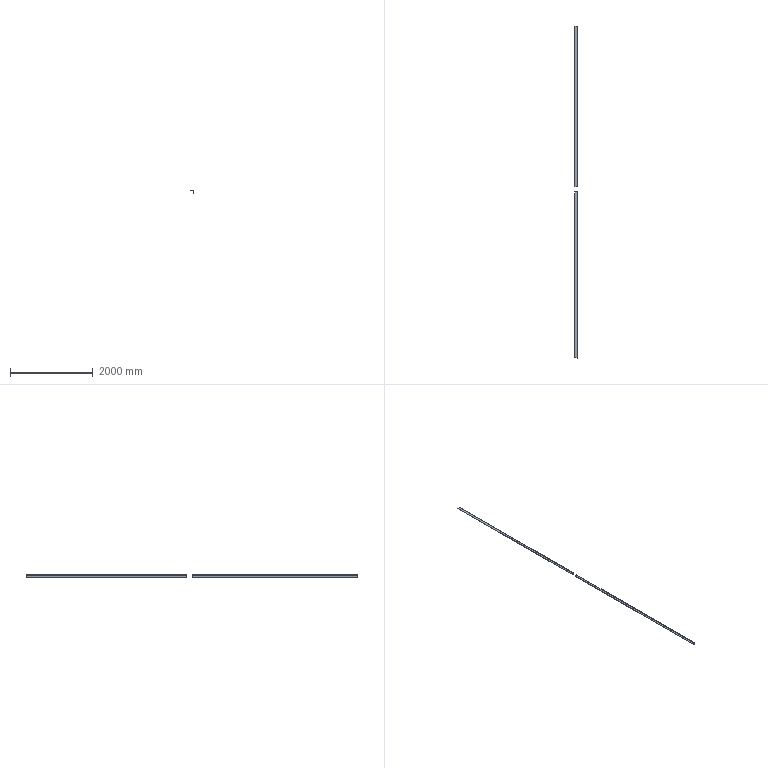Component | SolidWorks | 63#AngleIron-47 | 2 solids | 22 faces | box 63 x 8000 x 63 mm | volume 3919801 mm3 | plane 16 | cylinder 6 | commonest cylinder face diameters 2.667 x4 14 x2
STEP:
#1=CARTESIAN_POINT('',(81.493,-440.742,145.512));
#2=VERTEX_POINT('',#1);
#3=CARTESIAN_POINT('',(81.493,-598.222,145.512));
#4=VERTEX_POINT('',#3);
#5=CARTESIAN_POINT('',(81.493,-283.262,145.512));
#6=DIRECTION('',(-0.,-1.,0.));
#7=VECTOR('',#6,39.37);
#8=LINE('',#5,#7);
#9=EDGE_CURVE('',#2,#4,#8,.T.);
#10=ORIENTED_EDGE('',*,*,#9,.F.);
#11=CARTESIAN_POINT('',(81.493,-440.742,147.992));
#12=VERTEX_POINT('',#11);
#13=CARTESIAN_POINT('',(81.493,-440.742,145.512));
#14=DIRECTION('',(0.,-0.,1.));
#15=VECTOR('',#14,39.37);
#16=LINE('',#13,#15);
#17=EDGE_CURVE('',#2,#12,#16,.T.);
#18=ORIENTED_EDGE('',*,*,#17,.T.);
#19=CARTESIAN_POINT('',(81.493,-598.222,147.992));
#20=VERTEX_POINT('',#19);
#21=CARTESIAN_POINT('',(81.493,-283.262,147.992));
#22=DIRECTION('',(-0.,-1.,0.));
#23=VECTOR('',#22,39.37);
#24=LINE('',#21,#23);
#25=EDGE_CURVE('',#12,#20,#24,.T.);
#26=ORIENTED_EDGE('',*,*,#25,.T.);
#27=CARTESIAN_POINT('',(81.493,-598.222,145.512));
#28=DIRECTION('',(-0.,-0.,-1.));
#29=VECTOR('',#28,39.37);
#30=LINE('',#27,#29);
#31=EDGE_CURVE('',#20,#4,#30,.T.);
#32=ORIENTED_EDGE('',*,*,#31,.T.);
#33=EDGE_LOOP('',(#10,#18,#26,#32));
#34=FACE_OUTER_BOUND('',#33,.T.);
#35=CARTESIAN_POINT('',(81.493,-283.262,145.512));
#36=DIRECTION('',(-1.,0.,0.));
#37=DIRECTION('',(0.,1.,-0.));
#38=AXIS2_PLACEMENT_3D('',#35,#36,#37);
#39=PLANE('',#38);
#40=ADVANCED_FACE('',(#34),#39,.F.);
#41=CARTESIAN_POINT('',(81.388,-440.742,145.512));
#42=VERTEX_POINT('',#41);
#43=CARTESIAN_POINT('',(81.388,-598.222,145.512));
#44=VERTEX_POINT('',#43);
#45=CARTESIAN_POINT('',(81.388,-283.262,145.512));
#46=DIRECTION('',(-0.,-1.,0.));
#47=VECTOR('',#46,39.37);
#48=LINE('',#45,#47);
#49=EDGE_CURVE('',#42,#44,#48,.T.);
#50=ORIENTED_EDGE('',*,*,#49,.F.);
#51=CARTESIAN_POINT('',(81.493,-440.742,145.512));
#52=DIRECTION('',(1.,0.,-0.));
#53=VECTOR('',#52,39.37);
#54=LINE('',#51,#53);
#55=EDGE_CURVE('',#42,#2,#54,.T.);
#56=ORIENTED_EDGE('',*,*,#55,.T.);
#57=ORIENTED_EDGE('',*,*,#9,.T.);
#58=CARTESIAN_POINT('',(81.493,-598.222,145.512));
#59=DIRECTION('',(-1.,0.,0.));
#60=VECTOR('',#59,39.37);
#61=LINE('',#58,#60);
#62=EDGE_CURVE('',#4,#44,#61,.T.);
#63=ORIENTED_EDGE('',*,*,#62,.T.);
#64=EDGE_LOOP('',(#50,#56,#57,#63));
#65=FACE_OUTER_BOUND('',#64,.T.);
#66=CARTESIAN_POINT('',(81.493,-283.262,145.512));
#67=DIRECTION('',(0.,0.,1.));
#68=DIRECTION('',(1.,-0.,-0.));
#69=AXIS2_PLACEMENT_3D('',#66,#67,#68);
#70=PLANE('',#69);
#71=ADVANCED_FACE('',(#65),#70,.F.);
#72=CARTESIAN_POINT('',(81.336,-440.742,145.564));
#73=VERTEX_POINT('',#72);
#74=CARTESIAN_POINT('',(81.336,-598.222,145.564));
#75=VERTEX_POINT('',#74);
#76=CARTESIAN_POINT('',(81.336,-283.262,145.564));
#77=DIRECTION('',(-0.,-1.,0.));
#78=VECTOR('',#77,39.37);
#79=LINE('',#76,#78);
#80=EDGE_CURVE('',#73,#75,#79,.T.);
#81=ORIENTED_EDGE('',*,*,#80,.F.);
#82=CARTESIAN_POINT('',(81.388,-440.742,145.564));
#83=DIRECTION('',(0.,-1.,-0.));
#84=DIRECTION('',(-1.,0.,0.));
#85=AXIS2_PLACEMENT_3D('',#82,#83,#84);
#86=CIRCLE('',#85,0.05249);
#87=EDGE_CURVE('',#73,#42,#86,.T.);
#88=ORIENTED_EDGE('',*,*,#87,.T.);
#89=ORIENTED_EDGE('',*,*,#49,.T.);
#90=CARTESIAN_POINT('',(81.388,-598.222,145.564));
#91=DIRECTION('',(0.,1.,-0.));
#92=DIRECTION('',(1.,0.,0.));
#93=AXIS2_PLACEMENT_3D('',#90,#91,#92);
#94=CIRCLE('',#93,0.05249);
#95=EDGE_CURVE('',#44,#75,#94,.T.);
#96=ORIENTED_EDGE('',*,*,#95,.T.);
#97=EDGE_LOOP('',(#81,#88,#89,#96));
#98=FACE_OUTER_BOUND('',#97,.T.);
#99=CARTESIAN_POINT('',(81.388,-283.262,145.564));
#100=DIRECTION('',(-0.,-1.,0.));
#101=DIRECTION('',(-1.,0.,0.));
#102=AXIS2_PLACEMENT_3D('',#99,#100,#101);
#103=CYLINDRICAL_SURFACE('',#102,0.05249);
#104=ADVANCED_FACE('',(#98),#103,.T.);
#105=CARTESIAN_POINT('',(81.336,-440.742,147.559));
#106=VERTEX_POINT('',#105);
#107=CARTESIAN_POINT('',(81.336,-598.222,147.559));
#108=VERTEX_POINT('',#107);
#109=CARTESIAN_POINT('',(81.336,-283.262,147.559));
#110=DIRECTION('',(-0.,-1.,0.));
#111=VECTOR('',#110,39.37);
#112=LINE('',#109,#111);
#113=EDGE_CURVE('',#106,#108,#112,.T.);
#114=ORIENTED_EDGE('',*,*,#113,.F.);
#115=CARTESIAN_POINT('',(81.336,-440.742,147.559));
#116=DIRECTION('',(-0.,0.,-1.));
#117=VECTOR('',#116,39.37);
#118=LINE('',#115,#117);
#119=EDGE_CURVE('',#106,#73,#118,.T.);
#120=ORIENTED_EDGE('',*,*,#119,.T.);
#121=ORIENTED_EDGE('',*,*,#80,.T.);
#122=CARTESIAN_POINT('',(81.336,-598.222,147.559));
#123=DIRECTION('',(0.,0.,1.));
#124=VECTOR('',#123,39.37);
#125=LINE('',#122,#124);
#126=EDGE_CURVE('',#75,#108,#125,.T.);
#127=ORIENTED_EDGE('',*,*,#126,.T.);
#128=EDGE_LOOP('',(#114,#120,#121,#127));
#129=FACE_OUTER_BOUND('',#128,.T.);
#130=CARTESIAN_POINT('',(81.336,-283.262,147.559));
#131=DIRECTION('',(1.,-0.,-0.));
#132=DIRECTION('',(-0.,-0.,-1.));
#133=AXIS2_PLACEMENT_3D('',#130,#131,#132);
#134=PLANE('',#133);
#135=ADVANCED_FACE('',(#129),#134,.F.);
#136=CARTESIAN_POINT('',(81.06,-440.742,147.835));
#137=VERTEX_POINT('',#136);
#138=CARTESIAN_POINT('',(81.06,-598.222,147.835));
#139=VERTEX_POINT('',#138);
#140=CARTESIAN_POINT('',(81.06,-283.262,147.835));
#141=DIRECTION('',(-0.,-1.,0.));
#142=VECTOR('',#141,39.37);
#143=LINE('',#140,#142);
#144=EDGE_CURVE('',#137,#139,#143,.T.);
#145=ORIENTED_EDGE('',*,*,#144,.F.);
#146=CARTESIAN_POINT('',(81.06,-440.742,147.559));
#147=DIRECTION('',(0.,1.,0.));
#148=DIRECTION('',(-1.,0.,0.));
#149=AXIS2_PLACEMENT_3D('',#146,#147,#148);
#150=CIRCLE('',#149,0.2756);
#151=EDGE_CURVE('',#137,#106,#150,.T.);
#152=ORIENTED_EDGE('',*,*,#151,.T.);
#153=ORIENTED_EDGE('',*,*,#113,.T.);
#154=CARTESIAN_POINT('',(81.06,-598.222,147.559));
#155=DIRECTION('',(-0.,-1.,0.));
#156=DIRECTION('',(-1.,0.,0.));
#157=AXIS2_PLACEMENT_3D('',#154,#155,#156);
#158=CIRCLE('',#157,0.2756);
#159=EDGE_CURVE('',#108,#139,#158,.T.);
#160=ORIENTED_EDGE('',*,*,#159,.T.);
#161=EDGE_LOOP('',(#145,#152,#153,#160));
#162=FACE_OUTER_BOUND('',#161,.T.);
#163=CARTESIAN_POINT('',(81.06,-283.262,147.559));
#164=DIRECTION('',(-0.,-1.,0.));
#165=DIRECTION('',(-1.,0.,0.));
#166=AXIS2_PLACEMENT_3D('',#163,#164,#165);
#167=CYLINDRICAL_SURFACE('',#166,0.2756);
#168=ADVANCED_FACE('',(#162),#167,.F.);
#169=CARTESIAN_POINT('',(79.065,-440.742,147.835));
#170=VERTEX_POINT('',#169);
#171=CARTESIAN_POINT('',(79.065,-598.222,147.835));
#172=VERTEX_POINT('',#171);
#173=CARTESIAN_POINT('',(79.065,-283.262,147.835));
#174=DIRECTION('',(-0.,-1.,0.));
#175=VECTOR('',#174,39.37);
#176=LINE('',#173,#175);
#177=EDGE_CURVE('',#170,#172,#176,.T.);
#178=ORIENTED_EDGE('',*,*,#177,.F.);
#179=CARTESIAN_POINT('',(79.065,-440.742,147.835));
#180=DIRECTION('',(1.,0.,-0.));
#181=VECTOR('',#180,39.37);
#182=LINE('',#179,#181);
#183=EDGE_CURVE('',#170,#137,#182,.T.);
#184=ORIENTED_EDGE('',*,*,#183,.T.);
#185=ORIENTED_EDGE('',*,*,#144,.T.);
#186=CARTESIAN_POINT('',(79.065,-598.222,147.835));
#187=DIRECTION('',(-1.,0.,0.));
#188=VECTOR('',#187,39.37);
#189=LINE('',#186,#188);
#190=EDGE_CURVE('',#139,#172,#189,.T.);
#191=ORIENTED_EDGE('',*,*,#190,.T.);
#192=EDGE_LOOP('',(#178,#184,#185,#191));
#193=FACE_OUTER_BOUND('',#192,.T.);
#194=CARTESIAN_POINT('',(79.065,-283.262,147.835));
#195=DIRECTION('',(0.,0.,1.));
#196=DIRECTION('',(1.,-0.,-0.));
#197=AXIS2_PLACEMENT_3D('',#194,#195,#196);
#198=PLANE('',#197);
#199=ADVANCED_FACE('',(#193),#198,.F.);
#200=CARTESIAN_POINT('',(79.013,-440.742,147.887));
#201=VERTEX_POINT('',#200);
#202=CARTESIAN_POINT('',(79.013,-598.222,147.887));
#203=VERTEX_POINT('',#202);
#204=CARTESIAN_POINT('',(79.013,-283.262,147.887));
#205=DIRECTION('',(-0.,-1.,0.));
#206=VECTOR('',#205,39.37);
#207=LINE('',#204,#206);
#208=EDGE_CURVE('',#201,#203,#207,.T.);
#209=ORIENTED_EDGE('',*,*,#208,.F.);
#210=CARTESIAN_POINT('',(79.065,-440.742,147.887));
#211=DIRECTION('',(0.,-1.,-0.));
#212=DIRECTION('',(-1.,0.,0.));
#213=AXIS2_PLACEMENT_3D('',#210,#211,#212);
#214=CIRCLE('',#213,0.05249);
#215=EDGE_CURVE('',#201,#170,#214,.T.);
#216=ORIENTED_EDGE('',*,*,#215,.T.);
#217=ORIENTED_EDGE('',*,*,#177,.T.);
#218=CARTESIAN_POINT('',(79.065,-598.222,147.887));
#219=DIRECTION('',(0.,1.,-0.));
#220=DIRECTION('',(-1.,0.,0.));
#221=AXIS2_PLACEMENT_3D('',#218,#219,#220);
#222=CIRCLE('',#221,0.05249);
#223=EDGE_CURVE('',#172,#203,#222,.T.);
#224=ORIENTED_EDGE('',*,*,#223,.T.);
#225=EDGE_LOOP('',(#209,#216,#217,#224));
#226=FACE_OUTER_BOUND('',#225,.T.);
#227=CARTESIAN_POINT('',(79.065,-283.262,147.887));
#228=DIRECTION('',(-0.,-1.,0.));
#229=DIRECTION('',(-1.,0.,0.));
#230=AXIS2_PLACEMENT_3D('',#227,#228,#229);
#231=CYLINDRICAL_SURFACE('',#230,0.05249);
#232=ADVANCED_FACE('',(#226),#231,.T.);
#233=CARTESIAN_POINT('',(79.013,-440.742,147.992));
#234=VERTEX_POINT('',#233);
#235=CARTESIAN_POINT('',(79.013,-598.222,147.992));
#236=VERTEX_POINT('',#235);
#237=CARTESIAN_POINT('',(79.013,-283.262,147.992));
#238=DIRECTION('',(-0.,-1.,0.));
#239=VECTOR('',#238,39.37);
#240=LINE('',#237,#239);
#241=EDGE_CURVE('',#234,#236,#240,.T.);
#242=ORIENTED_EDGE('',*,*,#241,.F.);
#243=CARTESIAN_POINT('',(79.013,-440.742,147.992));
#244=DIRECTION('',(-0.,0.,-1.));
#245=VECTOR('',#244,39.37);
#246=LINE('',#243,#245);
#247=EDGE_CURVE('',#234,#201,#246,.T.);
#248=ORIENTED_EDGE('',*,*,#247,.T.);
#249=ORIENTED_EDGE('',*,*,#208,.T.);
#250=CARTESIAN_POINT('',(79.013,-598.222,147.992));
#251=DIRECTION('',(0.,0.,1.));
#252=VECTOR('',#251,39.37);
#253=LINE('',#250,#252);
#254=EDGE_CURVE('',#203,#236,#253,.T.);
#255=ORIENTED_EDGE('',*,*,#254,.T.);
#256=EDGE_LOOP('',(#242,#248,#249,#255));
#257=FACE_OUTER_BOUND('',#256,.T.);
#258=CARTESIAN_POINT('',(79.013,-283.262,147.992));
#259=DIRECTION('',(1.,-0.,-0.));
#260=DIRECTION('',(-0.,-1.,0.));
#261=AXIS2_PLACEMENT_3D('',#258,#259,#260);
#262=PLANE('',#261);
#263=ADVANCED_FACE('',(#257),#262,.F.);
#264=ORIENTED_EDGE('',*,*,#25,.F.);
#265=CARTESIAN_POINT('',(81.493,-440.742,147.992));
#266=DIRECTION('',(-1.,0.,0.));
#267=VECTOR('',#266,39.37);
#268=LINE('',#265,#267);
#269=EDGE_CURVE('',#12,#234,#268,.T.);
#270=ORIENTED_EDGE('',*,*,#269,.T.);
#271=ORIENTED_EDGE('',*,*,#241,.T.);
#272=CARTESIAN_POINT('',(81.493,-598.222,147.992));
#273=DIRECTION('',(1.,-0.,-0.));
#274=VECTOR('',#273,39.37);
#275=LINE('',#272,#274);
#276=EDGE_CURVE('',#236,#20,#275,.T.);
#277=ORIENTED_EDGE('',*,*,#276,.T.);
#278=EDGE_LOOP('',(#264,#270,#271,#277));
#279=FACE_OUTER_BOUND('',#278,.T.);
#280=CARTESIAN_POINT('',(81.493,-283.262,147.992));
#281=DIRECTION('',(-0.,-0.,-1.));
#282=DIRECTION('',(-1.,0.,0.));
#283=AXIS2_PLACEMENT_3D('',#280,#281,#282);
#284=PLANE('',#283);
#285=ADVANCED_FACE('',(#279),#284,.F.);
#286=ORIENTED_EDGE('',*,*,#31,.F.);
#287=ORIENTED_EDGE('',*,*,#276,.F.);
#288=ORIENTED_EDGE('',*,*,#254,.F.);
#289=ORIENTED_EDGE('',*,*,#223,.F.);
#290=ORIENTED_EDGE('',*,*,#190,.F.);
#291=ORIENTED_EDGE('',*,*,#159,.F.);
#292=ORIENTED_EDGE('',*,*,#126,.F.);
#293=ORIENTED_EDGE('',*,*,#95,.F.);
#294=ORIENTED_EDGE('',*,*,#62,.F.);
#295=EDGE_LOOP('',(#286,#287,#288,#289,#290,#291,#292,#293,#294));
#296=FACE_OUTER_BOUND('',#295,.T.);
#297=CARTESIAN_POINT('',(79.065,-598.222,147.887));
#298=DIRECTION('',(-0.,-1.,0.));
#299=DIRECTION('',(-1.,0.,0.));
#300=AXIS2_PLACEMENT_3D('',#297,#298,#299);
#301=PLANE('',#300);
#302=ADVANCED_FACE('',(#296),#301,.T.);
#303=ORIENTED_EDGE('',*,*,#55,.F.);
#304=ORIENTED_EDGE('',*,*,#87,.F.);
#305=ORIENTED_EDGE('',*,*,#119,.F.);
#306=ORIENTED_EDGE('',*,*,#151,.F.);
#307=ORIENTED_EDGE('',*,*,#183,.F.);
#308=ORIENTED_EDGE('',*,*,#215,.F.);
#309=ORIENTED_EDGE('',*,*,#247,.F.);
#310=ORIENTED_EDGE('',*,*,#269,.F.);
#311=ORIENTED_EDGE('',*,*,#17,.F.);
#312=EDGE_LOOP('',(#303,#304,#305,#306,#307,#308,#309,#310,#311));
#313=FACE_OUTER_BOUND('',#312,.T.);
#314=CARTESIAN_POINT('',(-68.113,-440.742,23.622));
#315=DIRECTION('',(0.,-1.,0.));
#316=DIRECTION('',(0.,-0.,-1.));
#317=AXIS2_PLACEMENT_3D('',#314,#315,#316);
#318=PLANE('',#317);
#319=ADVANCED_FACE('',(#313),#318,.F.);
#320=CLOSED_SHELL('',(#40,#71,#104,#135,#168,#199,#232,#263,#285,#302,#319));
#321=MANIFOLD_SOLID_BREP('',#320);
#322=CARTESIAN_POINT('',(81.493,-283.262,147.992));
#323=VERTEX_POINT('',#322);
#324=CARTESIAN_POINT('',(81.493,-283.262,145.512));
#325=VERTEX_POINT('',#324);
#326=CARTESIAN_POINT('',(81.493,-283.262,145.512));
#327=DIRECTION('',(-0.,-0.,-1.));
#328=VECTOR('',#327,39.37);
#329=LINE('',#326,#328);
#330=EDGE_CURVE('',#323,#325,#329,.T.);
#331=ORIENTED_EDGE('',*,*,#330,.T.);
#332=CARTESIAN_POINT('',(81.388,-283.262,145.512));
#333=VERTEX_POINT('',#332);
#334=CARTESIAN_POINT('',(81.493,-283.262,145.512));
#335=DIRECTION('',(-1.,0.,0.));
#336=VECTOR('',#335,39.37);
#337=LINE('',#334,#336);
#338=EDGE_CURVE('',#325,#333,#337,.T.);
#339=ORIENTED_EDGE('',*,*,#338,.T.);
#340=CARTESIAN_POINT('',(81.336,-283.262,145.564));
#341=VERTEX_POINT('',#340);
#342=CARTESIAN_POINT('',(81.388,-283.262,145.564));
#343=DIRECTION('',(0.,1.,-0.));
#344=DIRECTION('',(1.,0.,0.));
#345=AXIS2_PLACEMENT_3D('',#342,#343,#344);
#346=CIRCLE('',#345,0.05249);
#347=EDGE_CURVE('',#333,#341,#346,.T.);
#348=ORIENTED_EDGE('',*,*,#347,.T.);
#349=CARTESIAN_POINT('',(81.336,-283.262,147.559));
#350=VERTEX_POINT('',#349);
#351=CARTESIAN_POINT('',(81.336,-283.262,147.559));
#352=DIRECTION('',(0.,0.,1.));
#353=VECTOR('',#352,39.37);
#354=LINE('',#351,#353);
#355=EDGE_CURVE('',#341,#350,#354,.T.);
#356=ORIENTED_EDGE('',*,*,#355,.T.);
#357=CARTESIAN_POINT('',(81.06,-283.262,147.835));
#358=VERTEX_POINT('',#357);
#359=CARTESIAN_POINT('',(81.06,-283.262,147.559));
#360=DIRECTION('',(-0.,-1.,0.));
#361=DIRECTION('',(-1.,0.,0.));
#362=AXIS2_PLACEMENT_3D('',#359,#360,#361);
#363=CIRCLE('',#362,0.2756);
#364=EDGE_CURVE('',#350,#358,#363,.T.);
#365=ORIENTED_EDGE('',*,*,#364,.T.);
#366=CARTESIAN_POINT('',(79.065,-283.262,147.835));
#367=VERTEX_POINT('',#366);
#368=CARTESIAN_POINT('',(79.065,-283.262,147.835));
#369=DIRECTION('',(-1.,0.,0.));
#370=VECTOR('',#369,39.37);
#371=LINE('',#368,#370);
#372=EDGE_CURVE('',#358,#367,#371,.T.);
#373=ORIENTED_EDGE('',*,*,#372,.T.);
#374=CARTESIAN_POINT('',(79.013,-283.262,147.887));
#375=VERTEX_POINT('',#374);
#376=CARTESIAN_POINT('',(79.065,-283.262,147.887));
#377=DIRECTION('',(0.,1.,-0.));
#378=DIRECTION('',(-1.,0.,0.));
#379=AXIS2_PLACEMENT_3D('',#376,#377,#378);
#380=CIRCLE('',#379,0.05249);
#381=EDGE_CURVE('',#367,#375,#380,.T.);
#382=ORIENTED_EDGE('',*,*,#381,.T.);
#383=CARTESIAN_POINT('',(79.013,-283.262,147.992));
#384=VERTEX_POINT('',#383);
#385=CARTESIAN_POINT('',(79.013,-283.262,147.992));
#386=DIRECTION('',(0.,0.,1.));
#387=VECTOR('',#386,39.37);
#388=LINE('',#385,#387);
#389=EDGE_CURVE('',#375,#384,#388,.T.);
#390=ORIENTED_EDGE('',*,*,#389,.T.);
#391=CARTESIAN_POINT('',(81.493,-283.262,147.992));
#392=DIRECTION('',(1.,-0.,-0.));
#393=VECTOR('',#392,39.37);
#394=LINE('',#391,#393);
#395=EDGE_CURVE('',#384,#323,#394,.T.);
#396=ORIENTED_EDGE('',*,*,#395,.T.);
#397=EDGE_LOOP('',(#331,#339,#348,#356,#365,#373,#382,#390,#396));
#398=FACE_OUTER_BOUND('',#397,.T.);
#399=CARTESIAN_POINT('',(79.065,-283.262,147.887));
#400=DIRECTION('',(-0.,-1.,0.));
#401=DIRECTION('',(-1.,0.,0.));
#402=AXIS2_PLACEMENT_3D('',#399,#400,#401);
#403=PLANE('',#402);
#404=ADVANCED_FACE('',(#398),#403,.F.);
#405=CARTESIAN_POINT('',(79.013,-435.821,147.992));
#406=VERTEX_POINT('',#405);
#407=CARTESIAN_POINT('',(79.013,-283.262,147.992));
#408=DIRECTION('',(-0.,-1.,0.));
#409=VECTOR('',#408,39.37);
#410=LINE('',#407,#409);
#411=EDGE_CURVE('',#384,#406,#410,.T.);
#412=ORIENTED_EDGE('',*,*,#411,.T.);
#413=CARTESIAN_POINT('',(81.493,-435.821,147.992));
#414=VERTEX_POINT('',#413);
#415=CARTESIAN_POINT('',(81.493,-435.821,147.992));
#416=DIRECTION('',(1.,0.,-0.));
#417=VECTOR('',#416,39.37);
#418=LINE('',#415,#417);
#419=EDGE_CURVE('',#406,#414,#418,.T.);
#420=ORIENTED_EDGE('',*,*,#419,.T.);
#421=CARTESIAN_POINT('',(81.493,-283.262,147.992));
#422=DIRECTION('',(-0.,-1.,0.));
#423=VECTOR('',#422,39.37);
#424=LINE('',#421,#423);
#425=EDGE_CURVE('',#323,#414,#424,.T.);
#426=ORIENTED_EDGE('',*,*,#425,.F.);
#427=ORIENTED_EDGE('',*,*,#395,.F.);
#428=EDGE_LOOP('',(#412,#420,#426,#427));
#429=FACE_OUTER_BOUND('',#428,.T.);
#430=CARTESIAN_POINT('',(81.493,-283.262,147.992));
#431=DIRECTION('',(-0.,-0.,-1.));
#432=DIRECTION('',(-1.,0.,0.));
#433=AXIS2_PLACEMENT_3D('',#430,#431,#432);
#434=PLANE('',#433);
#435=ADVANCED_FACE('',(#429),#434,.F.);
#436=CARTESIAN_POINT('',(79.013,-435.821,147.887));
#437=VERTEX_POINT('',#436);
#438=CARTESIAN_POINT('',(79.013,-283.262,147.887));
#439=DIRECTION('',(-0.,-1.,0.));
#440=VECTOR('',#439,39.37);
#441=LINE('',#438,#440);
#442=EDGE_CURVE('',#375,#437,#441,.T.);
#443=ORIENTED_EDGE('',*,*,#442,.T.);
#444=CARTESIAN_POINT('',(79.013,-435.821,147.992));
#445=DIRECTION('',(0.,-0.,1.));
#446=VECTOR('',#445,39.37);
#447=LINE('',#444,#446);
#448=EDGE_CURVE('',#437,#406,#447,.T.);
#449=ORIENTED_EDGE('',*,*,#448,.T.);
#450=ORIENTED_EDGE('',*,*,#411,.F.);
#451=ORIENTED_EDGE('',*,*,#389,.F.);
#452=EDGE_LOOP('',(#443,#449,#450,#451));
#453=FACE_OUTER_BOUND('',#452,.T.);
#454=CARTESIAN_POINT('',(79.013,-283.262,147.992));
#455=DIRECTION('',(1.,-0.,-0.));
#456=DIRECTION('',(-0.,-1.,0.));
#457=AXIS2_PLACEMENT_3D('',#454,#455,#456);
#458=PLANE('',#457);
#459=ADVANCED_FACE('',(#453),#458,.F.);
#460=CARTESIAN_POINT('',(79.065,-435.821,147.835));
#461=VERTEX_POINT('',#460);
#462=CARTESIAN_POINT('',(79.065,-283.262,147.835));
#463=DIRECTION('',(-0.,-1.,0.));
#464=VECTOR('',#463,39.37);
#465=LINE('',#462,#464);
#466=EDGE_CURVE('',#367,#461,#465,.T.);
#467=ORIENTED_EDGE('',*,*,#466,.T.);
#468=CARTESIAN_POINT('',(79.065,-435.821,147.887));
#469=DIRECTION('',(0.,1.,0.));
#470=DIRECTION('',(1.,0.,0.));
#471=AXIS2_PLACEMENT_3D('',#468,#469,#470);
#472=CIRCLE('',#471,0.05249);
#473=EDGE_CURVE('',#461,#437,#472,.T.);
#474=ORIENTED_EDGE('',*,*,#473,.T.);
#475=ORIENTED_EDGE('',*,*,#442,.F.);
#476=ORIENTED_EDGE('',*,*,#381,.F.);
#477=EDGE_LOOP('',(#467,#474,#475,#476));
#478=FACE_OUTER_BOUND('',#477,.T.);
#479=CARTESIAN_POINT('',(79.065,-283.262,147.887));
#480=DIRECTION('',(-0.,-1.,0.));
#481=DIRECTION('',(-1.,0.,0.));
#482=AXIS2_PLACEMENT_3D('',#479,#480,#481);
#483=CYLINDRICAL_SURFACE('',#482,0.05249);
#484=ADVANCED_FACE('',(#478),#483,.T.);
#485=CARTESIAN_POINT('',(81.06,-435.821,147.835));
#486=VERTEX_POINT('',#485);
#487=CARTESIAN_POINT('',(81.06,-283.262,147.835));
#488=DIRECTION('',(-0.,-1.,0.));
#489=VECTOR('',#488,39.37);
#490=LINE('',#487,#489);
#491=EDGE_CURVE('',#358,#486,#490,.T.);
#492=ORIENTED_EDGE('',*,*,#491,.T.);
#493=CARTESIAN_POINT('',(79.065,-435.821,147.835));
#494=DIRECTION('',(-1.,0.,0.));
#495=VECTOR('',#494,39.37);
#496=LINE('',#493,#495);
#497=EDGE_CURVE('',#486,#461,#496,.T.);
#498=ORIENTED_EDGE('',*,*,#497,.T.);
#499=ORIENTED_EDGE('',*,*,#466,.F.);
#500=ORIENTED_EDGE('',*,*,#372,.F.);
#501=EDGE_LOOP('',(#492,#498,#499,#500));
#502=FACE_OUTER_BOUND('',#501,.T.);
#503=CARTESIAN_POINT('',(79.065,-283.262,147.835));
#504=DIRECTION('',(0.,0.,1.));
#505=DIRECTION('',(1.,-0.,-0.));
#506=AXIS2_PLACEMENT_3D('',#503,#504,#505);
#507=PLANE('',#506);
#508=ADVANCED_FACE('',(#502),#507,.F.);
#509=CARTESIAN_POINT('',(81.336,-435.821,147.559));
#510=VERTEX_POINT('',#509);
#511=CARTESIAN_POINT('',(81.336,-283.262,147.559));
#512=DIRECTION('',(-0.,-1.,0.));
#513=VECTOR('',#512,39.37);
#514=LINE('',#511,#513);
#515=EDGE_CURVE('',#350,#510,#514,.T.);
#516=ORIENTED_EDGE('',*,*,#515,.T.);
#517=CARTESIAN_POINT('',(81.06,-435.821,147.559));
#518=DIRECTION('',(0.,-1.,-0.));
#519=DIRECTION('',(1.,0.,0.));
#520=AXIS2_PLACEMENT_3D('',#517,#518,#519);
#521=CIRCLE('',#520,0.2756);
#522=EDGE_CURVE('',#510,#486,#521,.T.);
#523=ORIENTED_EDGE('',*,*,#522,.T.);
#524=ORIENTED_EDGE('',*,*,#491,.F.);
#525=ORIENTED_EDGE('',*,*,#364,.F.);
#526=EDGE_LOOP('',(#516,#523,#524,#525));
#527=FACE_OUTER_BOUND('',#526,.T.);
#528=CARTESIAN_POINT('',(81.06,-283.262,147.559));
#529=DIRECTION('',(-0.,-1.,0.));
#530=DIRECTION('',(-1.,0.,0.));
#531=AXIS2_PLACEMENT_3D('',#528,#529,#530);
#532=CYLINDRICAL_SURFACE('',#531,0.2756);
#533=ADVANCED_FACE('',(#527),#532,.F.);
#534=CARTESIAN_POINT('',(81.336,-435.821,145.564));
#535=VERTEX_POINT('',#534);
#536=CARTESIAN_POINT('',(81.336,-283.262,145.564));
#537=DIRECTION('',(-0.,-1.,0.));
#538=VECTOR('',#537,39.37);
#539=LINE('',#536,#538);
#540=EDGE_CURVE('',#341,#535,#539,.T.);
#541=ORIENTED_EDGE('',*,*,#540,.T.);
#542=CARTESIAN_POINT('',(81.336,-435.821,147.559));
#543=DIRECTION('',(0.,-0.,1.));
#544=VECTOR('',#543,39.37);
#545=LINE('',#542,#544);
#546=EDGE_CURVE('',#535,#510,#545,.T.);
#547=ORIENTED_EDGE('',*,*,#546,.T.);
#548=ORIENTED_EDGE('',*,*,#515,.F.);
#549=ORIENTED_EDGE('',*,*,#355,.F.);
#550=EDGE_LOOP('',(#541,#547,#548,#549));
#551=FACE_OUTER_BOUND('',#550,.T.);
#552=CARTESIAN_POINT('',(81.336,-283.262,147.559));
#553=DIRECTION('',(1.,-0.,-0.));
#554=DIRECTION('',(-0.,-0.,-1.));
#555=AXIS2_PLACEMENT_3D('',#552,#553,#554);
#556=PLANE('',#555);
#557=ADVANCED_FACE('',(#551),#556,.F.);
#558=CARTESIAN_POINT('',(81.388,-435.821,145.512));
#559=VERTEX_POINT('',#558);
#560=CARTESIAN_POINT('',(81.388,-283.262,145.512));
#561=DIRECTION('',(-0.,-1.,0.));
#562=VECTOR('',#561,39.37);
#563=LINE('',#560,#562);
#564=EDGE_CURVE('',#333,#559,#563,.T.);
#565=ORIENTED_EDGE('',*,*,#564,.T.);
#566=CARTESIAN_POINT('',(81.388,-435.821,145.564));
#567=DIRECTION('',(0.,1.,0.));
#568=DIRECTION('',(1.,0.,0.));
#569=AXIS2_PLACEMENT_3D('',#566,#567,#568);
#570=CIRCLE('',#569,0.05249);
#571=EDGE_CURVE('',#559,#535,#570,.T.);
#572=ORIENTED_EDGE('',*,*,#571,.T.);
#573=ORIENTED_EDGE('',*,*,#540,.F.);
#574=ORIENTED_EDGE('',*,*,#347,.F.);
#575=EDGE_LOOP('',(#565,#572,#573,#574));
#576=FACE_OUTER_BOUND('',#575,.T.);
#577=CARTESIAN_POINT('',(81.388,-283.262,145.564));
#578=DIRECTION('',(-0.,-1.,0.));
#579=DIRECTION('',(-1.,0.,0.));
#580=AXIS2_PLACEMENT_3D('',#577,#578,#579);
#581=CYLINDRICAL_SURFACE('',#580,0.05249);
#582=ADVANCED_FACE('',(#576),#581,.T.);
#583=CARTESIAN_POINT('',(81.493,-435.821,145.512));
#584=VERTEX_POINT('',#583);
#585=CARTESIAN_POINT('',(81.493,-283.262,145.512));
#586=DIRECTION('',(-0.,-1.,0.));
#587=VECTOR('',#586,39.37);
#588=LINE('',#585,#587);
#589=EDGE_CURVE('',#325,#584,#588,.T.);
#590=ORIENTED_EDGE('',*,*,#589,.T.);
#591=CARTESIAN_POINT('',(81.493,-435.821,145.512));
#592=DIRECTION('',(-1.,0.,0.));
#593=VECTOR('',#592,39.37);
#594=LINE('',#591,#593);
#595=EDGE_CURVE('',#584,#559,#594,.T.);
#596=ORIENTED_EDGE('',*,*,#595,.T.);
#597=ORIENTED_EDGE('',*,*,#564,.F.);
#598=ORIENTED_EDGE('',*,*,#338,.F.);
#599=EDGE_LOOP('',(#590,#596,#597,#598));
#600=FACE_OUTER_BOUND('',#599,.T.);
#601=CARTESIAN_POINT('',(81.493,-283.262,145.512));
#602=DIRECTION('',(0.,0.,1.));
#603=DIRECTION('',(1.,-0.,-0.));
#604=AXIS2_PLACEMENT_3D('',#601,#602,#603);
#605=PLANE('',#604);
#606=ADVANCED_FACE('',(#600),#605,.F.);
#607=ORIENTED_EDGE('',*,*,#425,.T.);
#608=CARTESIAN_POINT('',(81.493,-435.821,145.512));
#609=DIRECTION('',(-0.,0.,-1.));
#610=VECTOR('',#609,39.37);
#611=LINE('',#608,#610);
#612=EDGE_CURVE('',#414,#584,#611,.T.);
#613=ORIENTED_EDGE('',*,*,#612,.T.);
#614=ORIENTED_EDGE('',*,*,#589,.F.);
#615=ORIENTED_EDGE('',*,*,#330,.F.);
#616=EDGE_LOOP('',(#607,#613,#614,#615));
#617=FACE_OUTER_BOUND('',#616,.T.);
#618=CARTESIAN_POINT('',(81.493,-283.262,145.512));
#619=DIRECTION('',(-1.,0.,0.));
#620=DIRECTION('',(0.,1.,-0.));
#621=AXIS2_PLACEMENT_3D('',#618,#619,#620);
#622=PLANE('',#621);
#623=ADVANCED_FACE('',(#617),#622,.F.);
#624=ORIENTED_EDGE('',*,*,#419,.F.);
#625=ORIENTED_EDGE('',*,*,#448,.F.);
#626=ORIENTED_EDGE('',*,*,#473,.F.);
#627=ORIENTED_EDGE('',*,*,#497,.F.);
#628=ORIENTED_EDGE('',*,*,#522,.F.);
#629=ORIENTED_EDGE('',*,*,#546,.F.);
#630=ORIENTED_EDGE('',*,*,#571,.F.);
#631=ORIENTED_EDGE('',*,*,#595,.F.);
#632=ORIENTED_EDGE('',*,*,#612,.F.);
#633=EDGE_LOOP('',(#624,#625,#626,#627,#628,#629,#630,#631,#632));
#634=FACE_OUTER_BOUND('',#633,.T.);
#635=CARTESIAN_POINT('',(-68.113,-435.821,23.622));
#636=DIRECTION('',(0.,1.,-0.));
#637=DIRECTION('',(0.,0.,1.));
#638=AXIS2_PLACEMENT_3D('',#635,#636,#637);
#639=PLANE('',#638);
#640=ADVANCED_FACE('',(#634),#639,.F.);
#641=CLOSED_SHELL('',(#404,#435,#459,#484,#508,#533,#557,#582,#606,#623,#640));
#642=MANIFOLD_SOLID_BREP('',#641);
#643=CARTESIAN_POINT('',(0.,0.,0.));
#644=DIRECTION('',(0.,0.,1.));
#645=DIRECTION('',(1.,0.,0.));
#646=AXIS2_PLACEMENT_3D('',#643,#644,#645);
#647=(LENGTH_UNIT()NAMED_UNIT(*)SI_UNIT($,.METRE.));
#648=LENGTH_MEASURE_WITH_UNIT(LENGTH_MEASURE(0.0254),#647);
#649=DIMENSIONAL_EXPONENTS(1.,0.,0.,0.,0.,0.,0.);
#650=(CONVERSION_BASED_UNIT('',#648)LENGTH_UNIT()NAMED_UNIT(#649));
#651=UNCERTAINTY_MEASURE_WITH_UNIT(LENGTH_MEASURE(0.00001),#650,'','');
#652=(NAMED_UNIT(*)PLANE_ANGLE_UNIT()SI_UNIT($,.RADIAN.));
#653=(NAMED_UNIT(*)SI_UNIT($,.STERADIAN.)SOLID_ANGLE_UNIT());
#654=(GEOMETRIC_REPRESENTATION_CONTEXT(3)GLOBAL_UNCERTAINTY_ASSIGNED_CONTEXT((#651))GLOBAL_UNIT_ASSIGNED_CONTEXT((#650,#652,#653))REPRESENTATION_CONTEXT('',''));
#655=ADVANCED_BREP_SHAPE_REPRESENTATION('',(#321,#642,#646),#654);
#656=COLOUR_RGB('',0.7922,0.8196,0.9333);
#657=FILL_AREA_STYLE_COLOUR('',#656);
#658=FILL_AREA_STYLE('',(#657));
#659=SURFACE_STYLE_FILL_AREA(#658);
#660=SURFACE_SIDE_STYLE('',(#659));
#661=SURFACE_STYLE_USAGE(.BOTH.,#660);
#662=PRESENTATION_STYLE_ASSIGNMENT((#661));
#663=STYLED_ITEM('',(#662),#321);
#664=(LENGTH_UNIT()NAMED_UNIT(*)SI_UNIT($,.METRE.));
#665=LENGTH_MEASURE_WITH_UNIT(LENGTH_MEASURE(0.0254),#664);
#666=DIMENSIONAL_EXPONENTS(1.,0.,0.,0.,0.,0.,0.);
#667=(CONVERSION_BASED_UNIT('',#665)LENGTH_UNIT()NAMED_UNIT(#666));
#668=UNCERTAINTY_MEASURE_WITH_UNIT(LENGTH_MEASURE(0.00001),#667,'','');
#669=(NAMED_UNIT(*)PLANE_ANGLE_UNIT()SI_UNIT($,.RADIAN.));
#670=(NAMED_UNIT(*)SI_UNIT($,.STERADIAN.)SOLID_ANGLE_UNIT());
#671=(GEOMETRIC_REPRESENTATION_CONTEXT(3)GLOBAL_UNCERTAINTY_ASSIGNED_CONTEXT((#668))GLOBAL_UNIT_ASSIGNED_CONTEXT((#667,#669,#670))REPRESENTATION_CONTEXT('',''));
#672=MECHANICAL_DESIGN_GEOMETRIC_PRESENTATION_REPRESENTATION('',(#663),#671);
#673=PRESENTATION_LAYER_ASSIGNMENT('','',(#663));
#674=COLOUR_RGB('',0.7922,0.8196,0.9333);
#675=FILL_AREA_STYLE_COLOUR('',#674);
#676=FILL_AREA_STYLE('',(#675));
#677=SURFACE_STYLE_FILL_AREA(#676);
#678=SURFACE_SIDE_STYLE('',(#677));
#679=SURFACE_STYLE_USAGE(.BOTH.,#678);
#680=PRESENTATION_STYLE_ASSIGNMENT((#679));
#681=STYLED_ITEM('',(#680),#642);
#682=PRESENTATION_LAYER_ASSIGNMENT('','',(#681));
#683=(LENGTH_UNIT()NAMED_UNIT(*)SI_UNIT($,.METRE.));
#684=LENGTH_MEASURE_WITH_UNIT(LENGTH_MEASURE(0.0254),#683);
#685=DIMENSIONAL_EXPONENTS(1.,0.,0.,0.,0.,0.,0.);
#686=(CONVERSION_BASED_UNIT('',#684)LENGTH_UNIT()NAMED_UNIT(#685));
#687=UNCERTAINTY_MEASURE_WITH_UNIT(LENGTH_MEASURE(0.00001),#686,'','');
#688=(NAMED_UNIT(*)PLANE_ANGLE_UNIT()SI_UNIT($,.RADIAN.));
#689=(NAMED_UNIT(*)SI_UNIT($,.STERADIAN.)SOLID_ANGLE_UNIT());
#690=(GEOMETRIC_REPRESENTATION_CONTEXT(3)GLOBAL_UNCERTAINTY_ASSIGNED_CONTEXT((#687))GLOBAL_UNIT_ASSIGNED_CONTEXT((#686,#688,#689))REPRESENTATION_CONTEXT('',''));
#691=MECHANICAL_DESIGN_GEOMETRIC_PRESENTATION_REPRESENTATION('',(#681),#690);